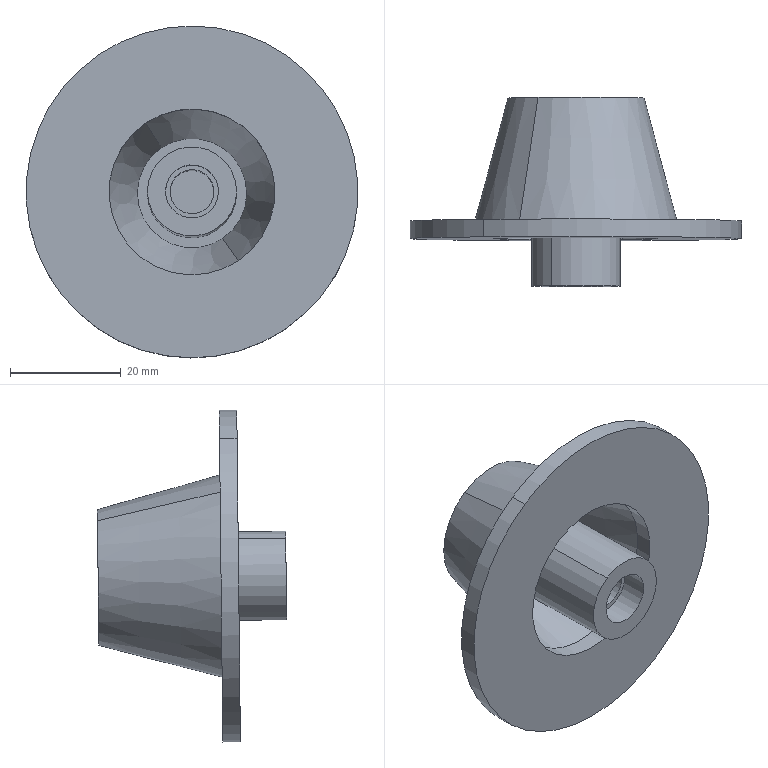Component | NX | SNAP_COVER | 2 solids | 20 faces | volume 19240 mm3 | cylinder 8 | plane 8 | cone 4 | commonest cylinder face diameters 30 x2 60 x2 16.129 x2 9.6 x1 7.938 x1